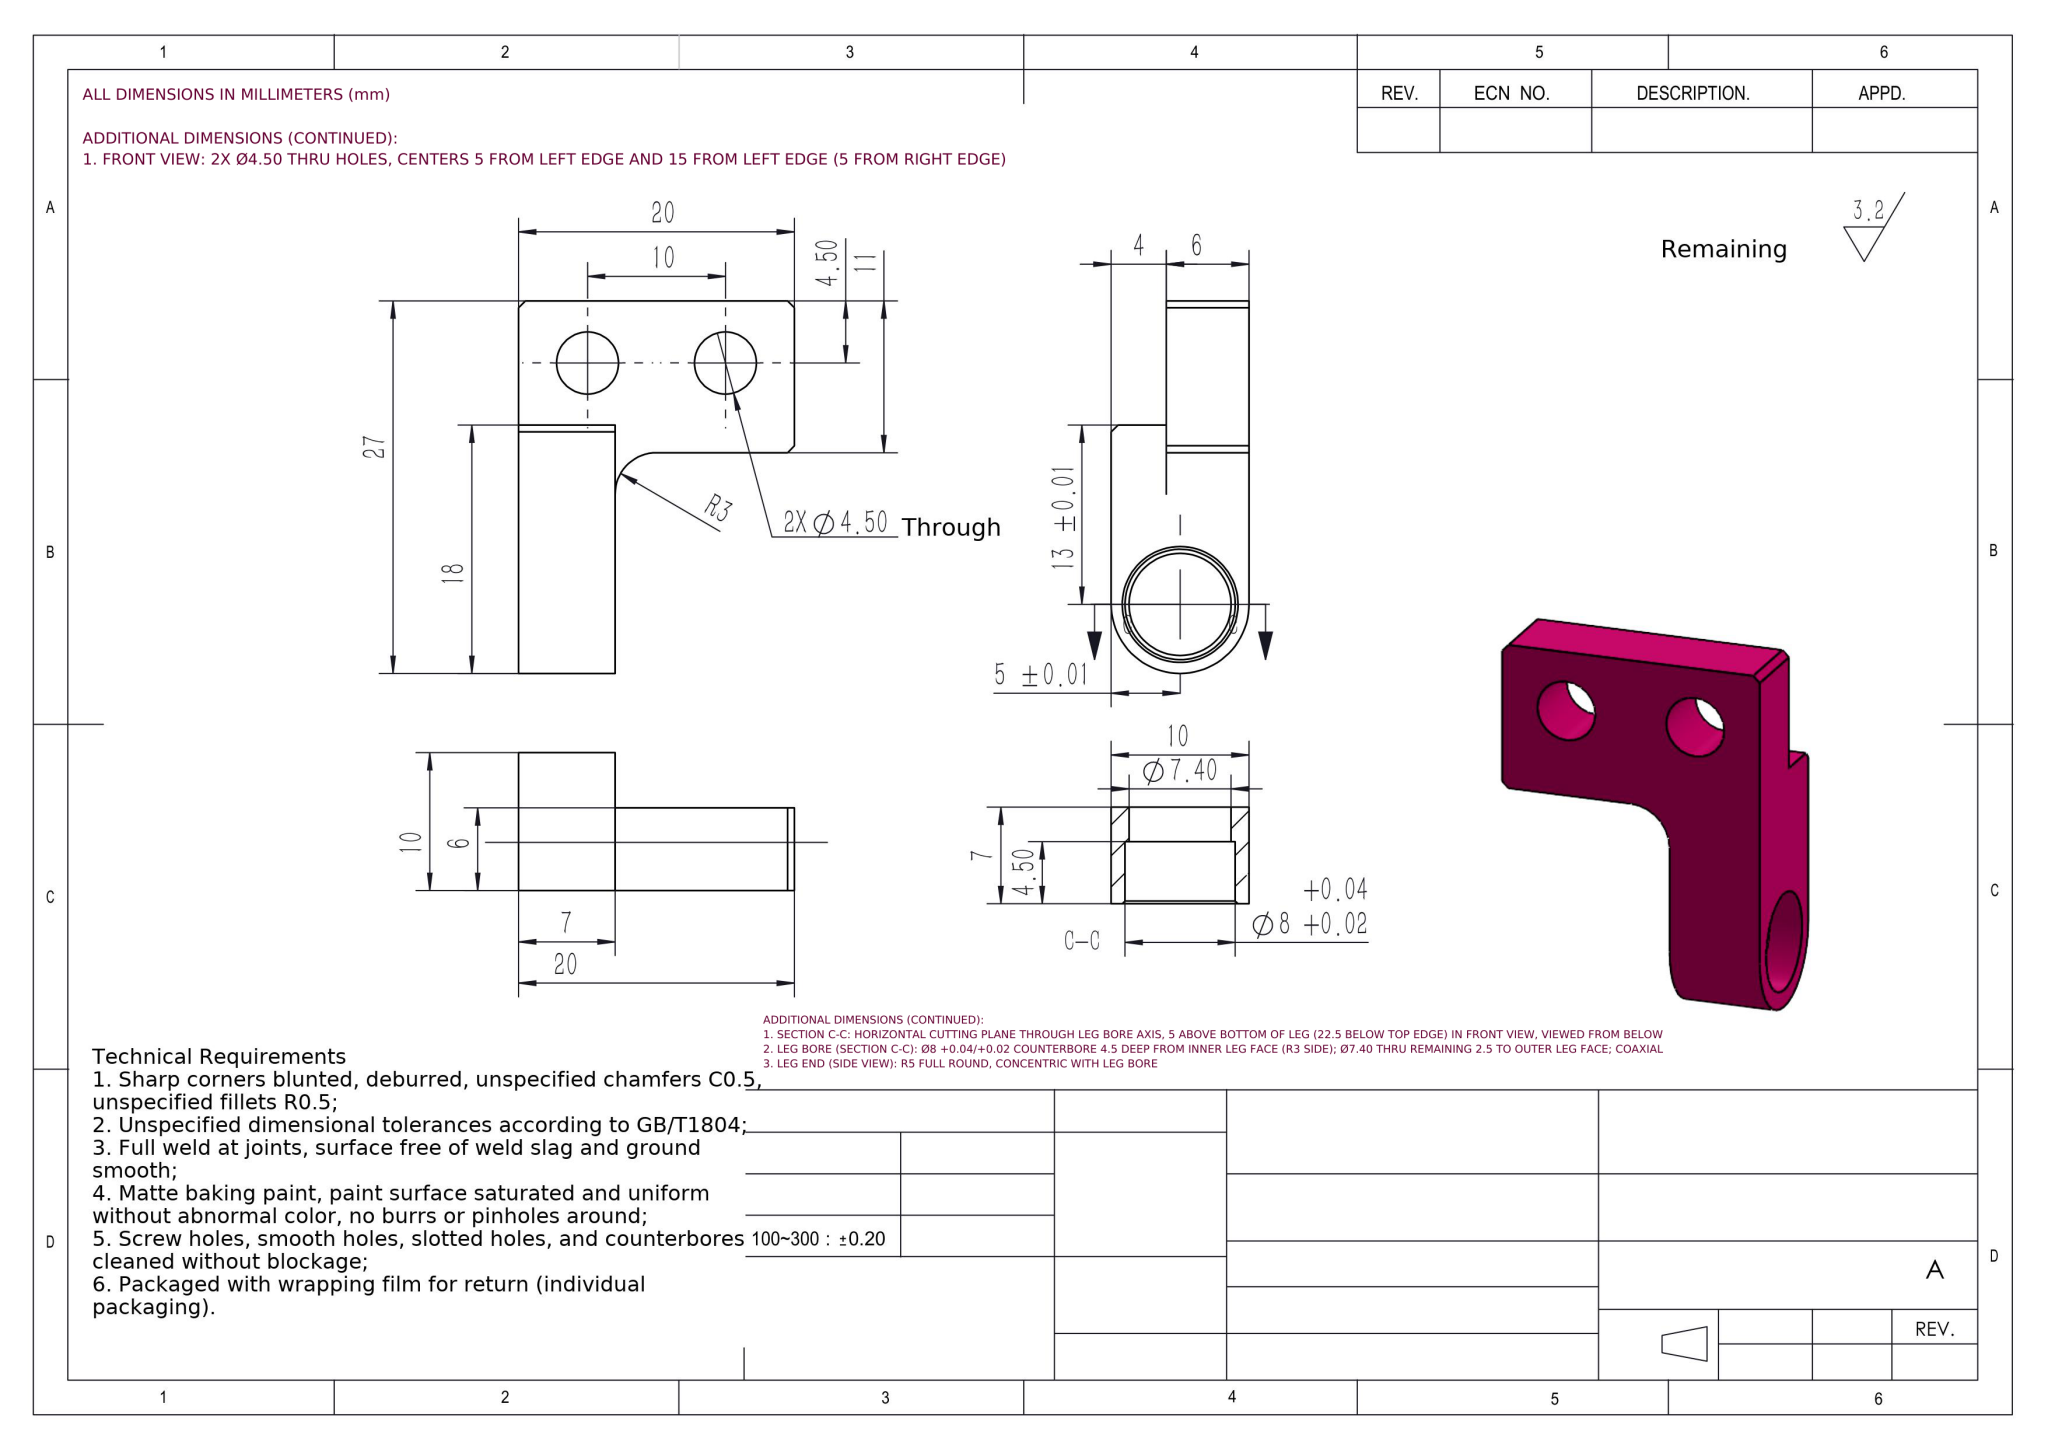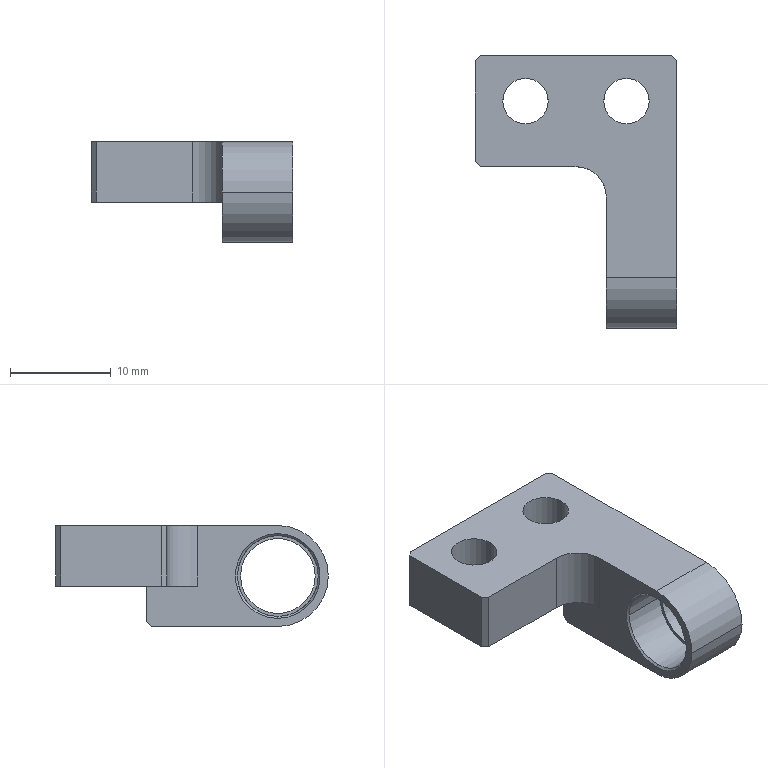Part | NX | mm | 1 solid | 27 faces | box 20 x 27 x 10 mm | volume 1904 mm3 | plane 14 | cylinder 11 | cone 2 | commonest cylinder face diameters 4.5 x4 8 x2 7.4 x2 10 x2 6 x1
STEP:
#1=COLOUR_RGB('',0.7922,0.8196,0.9333);
#2=FILL_AREA_STYLE_COLOUR('',#1);
#3=FILL_AREA_STYLE('',(#2));
#4=SURFACE_STYLE_FILL_AREA(#3);
#5=SURFACE_SIDE_STYLE('',(#4));
#6=SURFACE_STYLE_USAGE(.BOTH.,#5);
#7=PRESENTATION_STYLE_ASSIGNMENT((#6));
#8=CARTESIAN_POINT('',(3.2,-17.5,-6.));
#9=VERTEX_POINT('',#8);
#10=CARTESIAN_POINT('',(3.2,-21.5,-2.));
#11=VERTEX_POINT('',#10);
#12=CARTESIAN_POINT('',(3.2,-17.5,-2.));
#13=DIRECTION('',(-1.,0.,0.));
#14=DIRECTION('',(0.,0.,-1.));
#15=AXIS2_PLACEMENT_3D('',#12,#13,#14);
#16=CIRCLE('',#15,4.);
#17=EDGE_CURVE('',#9,#11,#16,.T.);
#18=ORIENTED_EDGE('',*,*,#17,.F.);
#19=CARTESIAN_POINT('',(3.,-17.5,-6.2));
#20=VERTEX_POINT('',#19);
#21=CARTESIAN_POINT('',(3.2,-17.5,-6.));
#22=DIRECTION('',(-0.7071,0.,-0.7071));
#23=VECTOR('',#22,1000.);
#24=LINE('',#21,#23);
#25=EDGE_CURVE('',#9,#20,#24,.T.);
#26=ORIENTED_EDGE('',*,*,#25,.T.);
#27=CARTESIAN_POINT('',(3.,-17.5,2.2));
#28=VERTEX_POINT('',#27);
#29=CARTESIAN_POINT('',(3.,-17.5,-2.));
#30=DIRECTION('',(1.,0.,0.));
#31=DIRECTION('',(-0.,1.,0.));
#32=AXIS2_PLACEMENT_3D('',#29,#30,#31);
#33=CIRCLE('',#32,4.2);
#34=EDGE_CURVE('',#28,#20,#33,.T.);
#35=ORIENTED_EDGE('',*,*,#34,.F.);
#36=CARTESIAN_POINT('',(3.2,-17.5,2.));
#37=VERTEX_POINT('',#36);
#38=CARTESIAN_POINT('',(3.2,-17.5,2.));
#39=DIRECTION('',(-0.7071,0.,0.7071));
#40=VECTOR('',#39,1000.);
#41=LINE('',#38,#40);
#42=EDGE_CURVE('',#37,#28,#41,.T.);
#43=ORIENTED_EDGE('',*,*,#42,.F.);
#44=CARTESIAN_POINT('',(3.2,-17.5,-2.));
#45=DIRECTION('',(-1.,0.,0.));
#46=DIRECTION('',(0.,0.,-1.));
#47=AXIS2_PLACEMENT_3D('',#44,#45,#46);
#48=CIRCLE('',#47,4.);
#49=EDGE_CURVE('',#11,#37,#48,.T.);
#50=ORIENTED_EDGE('',*,*,#49,.F.);
#51=EDGE_LOOP('',(#18,#26,#35,#43,#50));
#52=FACE_OUTER_BOUND('',#51,.T.);
#53=CARTESIAN_POINT('',(3.2,-17.5,-2.));
#54=DIRECTION('',(-1.,0.,0.));
#55=DIRECTION('',(0.,0.,1.));
#56=AXIS2_PLACEMENT_3D('',#53,#54,#55);
#57=CONICAL_SURFACE('',#56,4.,0.7854);
#58=ADVANCED_FACE('',(#52),#57,.F.);
#59=CARTESIAN_POINT('',(-2.75,0.,3.));
#60=VERTEX_POINT('',#59);
#61=CARTESIAN_POINT('',(-7.25,0.,3.));
#62=VERTEX_POINT('',#61);
#63=CARTESIAN_POINT('',(-5.,0.,3.));
#64=DIRECTION('',(0.,0.,-1.));
#65=DIRECTION('',(-1.,0.,0.));
#66=AXIS2_PLACEMENT_3D('',#63,#64,#65);
#67=CIRCLE('',#66,2.25);
#68=EDGE_CURVE('',#60,#62,#67,.T.);
#69=ORIENTED_EDGE('',*,*,#68,.F.);
#70=CARTESIAN_POINT('',(-2.75,0.,-3.));
#71=VERTEX_POINT('',#70);
#72=CARTESIAN_POINT('',(-2.75,0.,3.));
#73=DIRECTION('',(0.,0.,-1.));
#74=VECTOR('',#73,1000.);
#75=LINE('',#72,#74);
#76=EDGE_CURVE('',#60,#71,#75,.T.);
#77=ORIENTED_EDGE('',*,*,#76,.T.);
#78=CARTESIAN_POINT('',(-7.25,0.,-3.));
#79=VERTEX_POINT('',#78);
#80=CARTESIAN_POINT('',(-5.,0.,-3.));
#81=DIRECTION('',(0.,0.,-1.));
#82=DIRECTION('',(-1.,0.,0.));
#83=AXIS2_PLACEMENT_3D('',#80,#81,#82);
#84=CIRCLE('',#83,2.25);
#85=EDGE_CURVE('',#71,#79,#84,.T.);
#86=ORIENTED_EDGE('',*,*,#85,.T.);
#87=CARTESIAN_POINT('',(-7.25,0.,3.));
#88=DIRECTION('',(0.,0.,-1.));
#89=VECTOR('',#88,1000.);
#90=LINE('',#87,#89);
#91=EDGE_CURVE('',#62,#79,#90,.T.);
#92=ORIENTED_EDGE('',*,*,#91,.F.);
#93=EDGE_LOOP('',(#69,#77,#86,#92));
#94=FACE_OUTER_BOUND('',#93,.T.);
#95=CARTESIAN_POINT('',(-5.,0.,3.));
#96=DIRECTION('',(0.,0.,-1.));
#97=DIRECTION('',(-1.,0.,0.));
#98=AXIS2_PLACEMENT_3D('',#95,#96,#97);
#99=CYLINDRICAL_SURFACE('',#98,2.25);
#100=ADVANCED_FACE('',(#94),#99,.F.);
#101=CARTESIAN_POINT('',(7.25,-0.,3.));
#102=VERTEX_POINT('',#101);
#103=CARTESIAN_POINT('',(2.75,-0.,3.));
#104=VERTEX_POINT('',#103);
#105=CARTESIAN_POINT('',(5.,-0.,3.));
#106=DIRECTION('',(0.,0.,-1.));
#107=DIRECTION('',(-1.,0.,0.));
#108=AXIS2_PLACEMENT_3D('',#105,#106,#107);
#109=CIRCLE('',#108,2.25);
#110=EDGE_CURVE('',#102,#104,#109,.T.);
#111=ORIENTED_EDGE('',*,*,#110,.F.);
#112=CARTESIAN_POINT('',(7.25,-0.,-3.));
#113=VERTEX_POINT('',#112);
#114=CARTESIAN_POINT('',(7.25,-0.,3.));
#115=DIRECTION('',(0.,0.,-1.));
#116=VECTOR('',#115,1000.);
#117=LINE('',#114,#116);
#118=EDGE_CURVE('',#102,#113,#117,.T.);
#119=ORIENTED_EDGE('',*,*,#118,.T.);
#120=CARTESIAN_POINT('',(2.75,-0.,-3.));
#121=VERTEX_POINT('',#120);
#122=CARTESIAN_POINT('',(5.,-0.,-3.));
#123=DIRECTION('',(0.,0.,-1.));
#124=DIRECTION('',(-1.,0.,0.));
#125=AXIS2_PLACEMENT_3D('',#122,#123,#124);
#126=CIRCLE('',#125,2.25);
#127=EDGE_CURVE('',#113,#121,#126,.T.);
#128=ORIENTED_EDGE('',*,*,#127,.T.);
#129=CARTESIAN_POINT('',(2.75,-0.,3.));
#130=DIRECTION('',(0.,0.,-1.));
#131=VECTOR('',#130,1000.);
#132=LINE('',#129,#131);
#133=EDGE_CURVE('',#104,#121,#132,.T.);
#134=ORIENTED_EDGE('',*,*,#133,.F.);
#135=EDGE_LOOP('',(#111,#119,#128,#134));
#136=FACE_OUTER_BOUND('',#135,.T.);
#137=CARTESIAN_POINT('',(5.,-0.,3.));
#138=DIRECTION('',(0.,0.,-1.));
#139=DIRECTION('',(-1.,0.,0.));
#140=AXIS2_PLACEMENT_3D('',#137,#138,#139);
#141=CYLINDRICAL_SURFACE('',#140,2.25);
#142=ADVANCED_FACE('',(#136),#141,.F.);
#143=CARTESIAN_POINT('',(7.5,-13.5,-2.));
#144=VERTEX_POINT('',#143);
#145=CARTESIAN_POINT('',(7.5,-21.5,-2.));
#146=VERTEX_POINT('',#145);
#147=CARTESIAN_POINT('',(7.5,-17.5,-2.));
#148=DIRECTION('',(-1.,-0.,0.));
#149=DIRECTION('',(0.,-1.,0.));
#150=AXIS2_PLACEMENT_3D('',#147,#148,#149);
#151=CIRCLE('',#150,4.);
#152=EDGE_CURVE('',#144,#146,#151,.T.);
#153=ORIENTED_EDGE('',*,*,#152,.F.);
#154=CARTESIAN_POINT('',(3.2,-13.5,-2.));
#155=VERTEX_POINT('',#154);
#156=CARTESIAN_POINT('',(7.5,-13.5,-2.));
#157=DIRECTION('',(-1.,-0.,0.));
#158=VECTOR('',#157,1000.);
#159=LINE('',#156,#158);
#160=EDGE_CURVE('',#144,#155,#159,.T.);
#161=ORIENTED_EDGE('',*,*,#160,.T.);
#162=CARTESIAN_POINT('',(3.2,-17.5,-2.));
#163=DIRECTION('',(-1.,0.,0.));
#164=DIRECTION('',(0.,0.,-1.));
#165=AXIS2_PLACEMENT_3D('',#162,#163,#164);
#166=CIRCLE('',#165,4.);
#167=EDGE_CURVE('',#155,#9,#166,.T.);
#168=ORIENTED_EDGE('',*,*,#167,.T.);
#169=ORIENTED_EDGE('',*,*,#17,.T.);
#170=CARTESIAN_POINT('',(7.5,-21.5,-2.));
#171=DIRECTION('',(-1.,-0.,0.));
#172=VECTOR('',#171,1000.);
#173=LINE('',#170,#172);
#174=EDGE_CURVE('',#146,#11,#173,.T.);
#175=ORIENTED_EDGE('',*,*,#174,.F.);
#176=EDGE_LOOP('',(#153,#161,#168,#169,#175));
#177=FACE_OUTER_BOUND('',#176,.T.);
#178=CARTESIAN_POINT('',(7.5,-17.5,-2.));
#179=DIRECTION('',(-1.,-0.,0.));
#180=DIRECTION('',(0.,-1.,0.));
#181=AXIS2_PLACEMENT_3D('',#178,#179,#180);
#182=CYLINDRICAL_SURFACE('',#181,4.);
#183=ADVANCED_FACE('',(#177),#182,.F.);
#184=CARTESIAN_POINT('',(10.,-13.8,-2.));
#185=VERTEX_POINT('',#184);
#186=CARTESIAN_POINT('',(10.,-21.2,-2.));
#187=VERTEX_POINT('',#186);
#188=CARTESIAN_POINT('',(10.,-17.5,-2.));
#189=DIRECTION('',(-1.,-0.,0.));
#190=DIRECTION('',(0.,-1.,0.));
#191=AXIS2_PLACEMENT_3D('',#188,#189,#190);
#192=CIRCLE('',#191,3.7);
#193=EDGE_CURVE('',#185,#187,#192,.T.);
#194=ORIENTED_EDGE('',*,*,#193,.F.);
#195=CARTESIAN_POINT('',(7.5,-13.8,-2.));
#196=VERTEX_POINT('',#195);
#197=CARTESIAN_POINT('',(10.,-13.8,-2.));
#198=DIRECTION('',(-1.,-0.,0.));
#199=VECTOR('',#198,1000.);
#200=LINE('',#197,#199);
#201=EDGE_CURVE('',#185,#196,#200,.T.);
#202=ORIENTED_EDGE('',*,*,#201,.T.);
#203=CARTESIAN_POINT('',(7.5,-21.2,-2.));
#204=VERTEX_POINT('',#203);
#205=CARTESIAN_POINT('',(7.5,-17.5,-2.));
#206=DIRECTION('',(1.,0.,0.));
#207=DIRECTION('',(0.,-1.,0.));
#208=AXIS2_PLACEMENT_3D('',#205,#206,#207);
#209=CIRCLE('',#208,3.7);
#210=EDGE_CURVE('',#204,#196,#209,.T.);
#211=ORIENTED_EDGE('',*,*,#210,.F.);
#212=CARTESIAN_POINT('',(10.,-21.2,-2.));
#213=DIRECTION('',(-1.,-0.,0.));
#214=VECTOR('',#213,1000.);
#215=LINE('',#212,#214);
#216=EDGE_CURVE('',#187,#204,#215,.T.);
#217=ORIENTED_EDGE('',*,*,#216,.F.);
#218=EDGE_LOOP('',(#194,#202,#211,#217));
#219=FACE_OUTER_BOUND('',#218,.T.);
#220=CARTESIAN_POINT('',(10.,-17.5,-2.));
#221=DIRECTION('',(-1.,-0.,0.));
#222=DIRECTION('',(0.,-1.,0.));
#223=AXIS2_PLACEMENT_3D('',#220,#221,#222);
#224=CYLINDRICAL_SURFACE('',#223,3.7);
#225=ADVANCED_FACE('',(#219),#224,.F.);
#226=ORIENTED_EDGE('',*,*,#34,.T.);
#227=CARTESIAN_POINT('',(3.,-17.5,-2.));
#228=DIRECTION('',(1.,0.,0.));
#229=DIRECTION('',(-0.,1.,0.));
#230=AXIS2_PLACEMENT_3D('',#227,#228,#229);
#231=CIRCLE('',#230,4.2);
#232=EDGE_CURVE('',#20,#28,#231,.T.);
#233=ORIENTED_EDGE('',*,*,#232,.T.);
#234=EDGE_LOOP('',(#226,#233));
#235=FACE_BOUND('',#234,.T.);
#236=CARTESIAN_POINT('',(3.,-9.5,3.));
#237=VERTEX_POINT('',#236);
#238=CARTESIAN_POINT('',(3.,-17.5,3.));
#239=VERTEX_POINT('',#238);
#240=CARTESIAN_POINT('',(3.,-4.5,3.));
#241=DIRECTION('',(0.,-1.,-0.));
#242=VECTOR('',#241,1000.);
#243=LINE('',#240,#242);
#244=EDGE_CURVE('',#237,#239,#243,.T.);
#245=ORIENTED_EDGE('',*,*,#244,.F.);
#246=CARTESIAN_POINT('',(3.,-9.5,-3.));
#247=VERTEX_POINT('',#246);
#248=CARTESIAN_POINT('',(3.,-9.5,-3.));
#249=DIRECTION('',(0.,0.,-1.));
#250=VECTOR('',#249,1000.);
#251=LINE('',#248,#250);
#252=EDGE_CURVE('',#237,#247,#251,.T.);
#253=ORIENTED_EDGE('',*,*,#252,.T.);
#254=CARTESIAN_POINT('',(3.,-4.5,-3.));
#255=VERTEX_POINT('',#254);
#256=CARTESIAN_POINT('',(3.,-6.5,-3.));
#257=DIRECTION('',(0.,1.,0.));
#258=VECTOR('',#257,1000.);
#259=LINE('',#256,#258);
#260=EDGE_CURVE('',#247,#255,#259,.T.);
#261=ORIENTED_EDGE('',*,*,#260,.T.);
#262=CARTESIAN_POINT('',(3.,-4.5,-6.5));
#263=VERTEX_POINT('',#262);
#264=CARTESIAN_POINT('',(3.,-4.5,3.));
#265=DIRECTION('',(0.,0.,1.));
#266=VECTOR('',#265,1000.);
#267=LINE('',#264,#266);
#268=EDGE_CURVE('',#263,#255,#267,.T.);
#269=ORIENTED_EDGE('',*,*,#268,.F.);
#270=CARTESIAN_POINT('',(3.,-5.,-7.));
#271=VERTEX_POINT('',#270);
#272=CARTESIAN_POINT('',(3.,-5.,-7.));
#273=DIRECTION('',(0.,-0.7071,-0.7071));
#274=VECTOR('',#273,1000.);
#275=LINE('',#272,#274);
#276=EDGE_CURVE('',#263,#271,#275,.T.);
#277=ORIENTED_EDGE('',*,*,#276,.T.);
#278=CARTESIAN_POINT('',(3.,-17.5,-7.));
#279=VERTEX_POINT('',#278);
#280=CARTESIAN_POINT('',(3.,-4.5,-7.));
#281=DIRECTION('',(-0.,1.,0.));
#282=VECTOR('',#281,1000.);
#283=LINE('',#280,#282);
#284=EDGE_CURVE('',#279,#271,#283,.T.);
#285=ORIENTED_EDGE('',*,*,#284,.F.);
#286=CARTESIAN_POINT('',(3.,-22.5,-2.));
#287=VERTEX_POINT('',#286);
#288=CARTESIAN_POINT('',(3.,-17.5,-2.));
#289=DIRECTION('',(-1.,-0.,0.));
#290=DIRECTION('',(-0.,1.,0.));
#291=AXIS2_PLACEMENT_3D('',#288,#289,#290);
#292=CIRCLE('',#291,5.);
#293=EDGE_CURVE('',#279,#287,#292,.T.);
#294=ORIENTED_EDGE('',*,*,#293,.T.);
#295=CARTESIAN_POINT('',(3.,-17.5,-2.));
#296=DIRECTION('',(-1.,-0.,0.));
#297=DIRECTION('',(-0.,1.,0.));
#298=AXIS2_PLACEMENT_3D('',#295,#296,#297);
#299=CIRCLE('',#298,5.);
#300=EDGE_CURVE('',#287,#239,#299,.T.);
#301=ORIENTED_EDGE('',*,*,#300,.T.);
#302=EDGE_LOOP('',(#245,#253,#261,#269,#277,#285,#294,#301));
#303=FACE_OUTER_BOUND('',#302,.T.);
#304=CARTESIAN_POINT('',(3.,0.,0.));
#305=DIRECTION('',(1.,0.,0.));
#306=DIRECTION('',(-0.,1.,0.));
#307=AXIS2_PLACEMENT_3D('',#304,#305,#306);
#308=PLANE('',#307);
#309=ADVANCED_FACE('',(#235,#303),#308,.F.);
#310=ORIENTED_EDGE('',*,*,#201,.F.);
#311=CARTESIAN_POINT('',(10.,-17.5,-2.));
#312=DIRECTION('',(-1.,-0.,0.));
#313=DIRECTION('',(0.,-1.,0.));
#314=AXIS2_PLACEMENT_3D('',#311,#312,#313);
#315=CIRCLE('',#314,3.7);
#316=EDGE_CURVE('',#187,#185,#315,.T.);
#317=ORIENTED_EDGE('',*,*,#316,.F.);
#318=ORIENTED_EDGE('',*,*,#216,.T.);
#319=CARTESIAN_POINT('',(7.5,-17.5,-2.));
#320=DIRECTION('',(1.,0.,0.));
#321=DIRECTION('',(0.,-1.,0.));
#322=AXIS2_PLACEMENT_3D('',#319,#320,#321);
#323=CIRCLE('',#322,3.7);
#324=EDGE_CURVE('',#196,#204,#323,.T.);
#325=ORIENTED_EDGE('',*,*,#324,.F.);
#326=EDGE_LOOP('',(#310,#317,#318,#325));
#327=FACE_OUTER_BOUND('',#326,.T.);
#328=CARTESIAN_POINT('',(10.,-17.5,-2.));
#329=DIRECTION('',(-1.,-0.,0.));
#330=DIRECTION('',(0.,-1.,0.));
#331=AXIS2_PLACEMENT_3D('',#328,#329,#330);
#332=CYLINDRICAL_SURFACE('',#331,3.7);
#333=ADVANCED_FACE('',(#327),#332,.F.);
#334=ORIENTED_EDGE('',*,*,#316,.T.);
#335=ORIENTED_EDGE('',*,*,#193,.T.);
#336=EDGE_LOOP('',(#334,#335));
#337=FACE_BOUND('',#336,.T.);
#338=CARTESIAN_POINT('',(10.,-17.5,-7.));
#339=VERTEX_POINT('',#338);
#340=CARTESIAN_POINT('',(10.,-5.,-7.));
#341=VERTEX_POINT('',#340);
#342=CARTESIAN_POINT('',(10.,-4.5,-7.));
#343=DIRECTION('',(-0.,1.,0.));
#344=VECTOR('',#343,1000.);
#345=LINE('',#342,#344);
#346=EDGE_CURVE('',#339,#341,#345,.T.);
#347=ORIENTED_EDGE('',*,*,#346,.T.);
#348=CARTESIAN_POINT('',(10.,-4.5,-6.5));
#349=VERTEX_POINT('',#348);
#350=CARTESIAN_POINT('',(10.,-5.,-7.));
#351=DIRECTION('',(0.,0.7071,0.7071));
#352=VECTOR('',#351,1000.);
#353=LINE('',#350,#352);
#354=EDGE_CURVE('',#341,#349,#353,.T.);
#355=ORIENTED_EDGE('',*,*,#354,.T.);
#356=CARTESIAN_POINT('',(10.,-4.5,-3.));
#357=VERTEX_POINT('',#356);
#358=CARTESIAN_POINT('',(10.,-4.5,3.));
#359=DIRECTION('',(0.,0.,1.));
#360=VECTOR('',#359,1000.);
#361=LINE('',#358,#360);
#362=EDGE_CURVE('',#349,#357,#361,.T.);
#363=ORIENTED_EDGE('',*,*,#362,.T.);
#364=CARTESIAN_POINT('',(10.,4.,-3.));
#365=VERTEX_POINT('',#364);
#366=CARTESIAN_POINT('',(10.,4.5,-3.));
#367=DIRECTION('',(0.,1.,0.));
#368=VECTOR('',#367,1000.);
#369=LINE('',#366,#368);
#370=EDGE_CURVE('',#357,#365,#369,.T.);
#371=ORIENTED_EDGE('',*,*,#370,.T.);
#372=CARTESIAN_POINT('',(10.,4.,3.));
#373=VERTEX_POINT('',#372);
#374=CARTESIAN_POINT('',(10.,4.,3.));
#375=DIRECTION('',(0.,0.,1.));
#376=VECTOR('',#375,1000.);
#377=LINE('',#374,#376);
#378=EDGE_CURVE('',#365,#373,#377,.T.);
#379=ORIENTED_EDGE('',*,*,#378,.T.);
#380=CARTESIAN_POINT('',(10.,-17.5,3.));
#381=VERTEX_POINT('',#380);
#382=CARTESIAN_POINT('',(10.,4.5,3.));
#383=DIRECTION('',(0.,1.,0.));
#384=VECTOR('',#383,1000.);
#385=LINE('',#382,#384);
#386=EDGE_CURVE('',#381,#373,#385,.T.);
#387=ORIENTED_EDGE('',*,*,#386,.F.);
#388=CARTESIAN_POINT('',(10.,-22.5,-2.));
#389=VERTEX_POINT('',#388);
#390=CARTESIAN_POINT('',(10.,-17.5,-2.));
#391=DIRECTION('',(1.,0.,0.));
#392=DIRECTION('',(0.,0.,1.));
#393=AXIS2_PLACEMENT_3D('',#390,#391,#392);
#394=CIRCLE('',#393,5.);
#395=EDGE_CURVE('',#381,#389,#394,.T.);
#396=ORIENTED_EDGE('',*,*,#395,.T.);
#397=CARTESIAN_POINT('',(10.,-17.5,-2.));
#398=DIRECTION('',(1.,0.,0.));
#399=DIRECTION('',(0.,0.,1.));
#400=AXIS2_PLACEMENT_3D('',#397,#398,#399);
#401=CIRCLE('',#400,5.);
#402=EDGE_CURVE('',#389,#339,#401,.T.);
#403=ORIENTED_EDGE('',*,*,#402,.T.);
#404=EDGE_LOOP('',(#347,#355,#363,#371,#379,#387,#396,#403));
#405=FACE_OUTER_BOUND('',#404,.T.);
#406=CARTESIAN_POINT('',(10.,4.5,3.));
#407=DIRECTION('',(-1.,0.,0.));
#408=DIRECTION('',(0.,0.,1.));
#409=AXIS2_PLACEMENT_3D('',#406,#407,#408);
#410=PLANE('',#409);
#411=ADVANCED_FACE('',(#337,#405),#410,.F.);
#412=CARTESIAN_POINT('',(9.5,4.5,3.));
#413=VERTEX_POINT('',#412);
#414=CARTESIAN_POINT('',(-9.5,4.5,3.));
#415=VERTEX_POINT('',#414);
#416=CARTESIAN_POINT('',(-10.,4.5,3.));
#417=DIRECTION('',(-1.,0.,0.));
#418=VECTOR('',#417,1000.);
#419=LINE('',#416,#418);
#420=EDGE_CURVE('',#413,#415,#419,.T.);
#421=ORIENTED_EDGE('',*,*,#420,.F.);
#422=CARTESIAN_POINT('',(9.5,4.5,-3.));
#423=VERTEX_POINT('',#422);
#424=CARTESIAN_POINT('',(9.5,4.5,3.));
#425=DIRECTION('',(0.,0.,-1.));
#426=VECTOR('',#425,1000.);
#427=LINE('',#424,#426);
#428=EDGE_CURVE('',#413,#423,#427,.T.);
#429=ORIENTED_EDGE('',*,*,#428,.T.);
#430=CARTESIAN_POINT('',(-9.5,4.5,-3.));
#431=VERTEX_POINT('',#430);
#432=CARTESIAN_POINT('',(-10.,4.5,-3.));
#433=DIRECTION('',(-1.,0.,0.));
#434=VECTOR('',#433,1000.);
#435=LINE('',#432,#434);
#436=EDGE_CURVE('',#423,#431,#435,.T.);
#437=ORIENTED_EDGE('',*,*,#436,.T.);
#438=CARTESIAN_POINT('',(-9.5,4.5,3.));
#439=DIRECTION('',(0.,0.,1.));
#440=VECTOR('',#439,1000.);
#441=LINE('',#438,#440);
#442=EDGE_CURVE('',#431,#415,#441,.T.);
#443=ORIENTED_EDGE('',*,*,#442,.T.);
#444=EDGE_LOOP('',(#421,#429,#437,#443));
#445=FACE_OUTER_BOUND('',#444,.T.);
#446=CARTESIAN_POINT('',(-10.,4.5,3.));
#447=DIRECTION('',(0.,-1.,0.));
#448=DIRECTION('',(0.,0.,-1.));
#449=AXIS2_PLACEMENT_3D('',#446,#447,#448);
#450=PLANE('',#449);
#451=ADVANCED_FACE('',(#445),#450,.F.);
#452=CARTESIAN_POINT('',(-10.,4.,-3.));
#453=VERTEX_POINT('',#452);
#454=CARTESIAN_POINT('',(-10.,-6.,-3.));
#455=VERTEX_POINT('',#454);
#456=CARTESIAN_POINT('',(-10.,4.5,-3.));
#457=DIRECTION('',(0.,-1.,0.));
#458=VECTOR('',#457,1000.);
#459=LINE('',#456,#458);
#460=EDGE_CURVE('',#453,#455,#459,.T.);
#461=ORIENTED_EDGE('',*,*,#460,.T.);
#462=CARTESIAN_POINT('',(-10.,-6.,3.));
#463=VERTEX_POINT('',#462);
#464=CARTESIAN_POINT('',(-10.,-6.,3.));
#465=DIRECTION('',(0.,0.,1.));
#466=VECTOR('',#465,1000.);
#467=LINE('',#464,#466);
#468=EDGE_CURVE('',#455,#463,#467,.T.);
#469=ORIENTED_EDGE('',*,*,#468,.T.);
#470=CARTESIAN_POINT('',(-10.,4.,3.));
#471=VERTEX_POINT('',#470);
#472=CARTESIAN_POINT('',(-10.,4.5,3.));
#473=DIRECTION('',(0.,-1.,0.));
#474=VECTOR('',#473,1000.);
#475=LINE('',#472,#474);
#476=EDGE_CURVE('',#471,#463,#475,.T.);
#477=ORIENTED_EDGE('',*,*,#476,.F.);
#478=CARTESIAN_POINT('',(-10.,4.,3.));
#479=DIRECTION('',(0.,0.,-1.));
#480=VECTOR('',#479,1000.);
#481=LINE('',#478,#480);
#482=EDGE_CURVE('',#471,#453,#481,.T.);
#483=ORIENTED_EDGE('',*,*,#482,.T.);
#484=EDGE_LOOP('',(#461,#469,#477,#483));
#485=FACE_OUTER_BOUND('',#484,.T.);
#486=CARTESIAN_POINT('',(-10.,4.5,3.));
#487=DIRECTION('',(1.,0.,0.));
#488=DIRECTION('',(0.,0.,-1.));
#489=AXIS2_PLACEMENT_3D('',#486,#487,#488);
#490=PLANE('',#489);
#491=ADVANCED_FACE('',(#485),#490,.F.);
#492=CARTESIAN_POINT('',(-5.,0.,3.));
#493=DIRECTION('',(0.,0.,-1.));
#494=DIRECTION('',(-1.,0.,0.));
#495=AXIS2_PLACEMENT_3D('',#492,#493,#494);
#496=CIRCLE('',#495,2.25);
#497=EDGE_CURVE('',#62,#60,#496,.T.);
#498=ORIENTED_EDGE('',*,*,#497,.T.);
#499=ORIENTED_EDGE('',*,*,#68,.T.);
#500=EDGE_LOOP('',(#498,#499));
#501=FACE_BOUND('',#500,.T.);
#502=CARTESIAN_POINT('',(5.,-0.,3.));
#503=DIRECTION('',(0.,0.,-1.));
#504=DIRECTION('',(-1.,0.,0.));
#505=AXIS2_PLACEMENT_3D('',#502,#503,#504);
#506=CIRCLE('',#505,2.25);
#507=EDGE_CURVE('',#104,#102,#506,.T.);
#508=ORIENTED_EDGE('',*,*,#507,.T.);
#509=ORIENTED_EDGE('',*,*,#110,.T.);
#510=EDGE_LOOP('',(#508,#509));
#511=FACE_BOUND('',#510,.T.);
#512=ORIENTED_EDGE('',*,*,#476,.T.);
#513=CARTESIAN_POINT('',(-9.5,-6.5,3.));
#514=VERTEX_POINT('',#513);
#515=CARTESIAN_POINT('',(-8.,-8.,3.));
#516=DIRECTION('',(0.7071,-0.7071,0.));
#517=VECTOR('',#516,1000.);
#518=LINE('',#515,#517);
#519=EDGE_CURVE('',#463,#514,#518,.T.);
#520=ORIENTED_EDGE('',*,*,#519,.T.);
#521=CARTESIAN_POINT('',(0.,-6.5,3.));
#522=VERTEX_POINT('',#521);
#523=CARTESIAN_POINT('',(3.,-6.5,3.));
#524=DIRECTION('',(-1.,0.,-0.));
#525=VECTOR('',#524,1000.);
#526=LINE('',#523,#525);
#527=EDGE_CURVE('',#522,#514,#526,.T.);
#528=ORIENTED_EDGE('',*,*,#527,.F.);
#529=CARTESIAN_POINT('',(0.,-9.5,3.));
#530=DIRECTION('',(0.,0.,-1.));
#531=DIRECTION('',(1.,0.,0.));
#532=AXIS2_PLACEMENT_3D('',#529,#530,#531);
#533=CIRCLE('',#532,3.);
#534=EDGE_CURVE('',#522,#237,#533,.T.);
#535=ORIENTED_EDGE('',*,*,#534,.T.);
#536=ORIENTED_EDGE('',*,*,#244,.T.);
#537=CARTESIAN_POINT('',(0.,-17.5,3.));
#538=DIRECTION('',(1.,0.,0.));
#539=VECTOR('',#538,1000.);
#540=LINE('',#537,#539);
#541=EDGE_CURVE('',#239,#381,#540,.T.);
#542=ORIENTED_EDGE('',*,*,#541,.T.);
#543=ORIENTED_EDGE('',*,*,#386,.T.);
#544=CARTESIAN_POINT('',(7.,7.,3.));
#545=DIRECTION('',(-0.7071,0.7071,0.));
#546=VECTOR('',#545,1000.);
#547=LINE('',#544,#546);
#548=EDGE_CURVE('',#373,#413,#547,.T.);
#549=ORIENTED_EDGE('',*,*,#548,.T.);
#550=ORIENTED_EDGE('',*,*,#420,.T.);
#551=CARTESIAN_POINT('',(-7.,7.,3.));
#552=DIRECTION('',(-0.7071,-0.7071,0.));
#553=VECTOR('',#552,1000.);
#554=LINE('',#551,#553);
#555=EDGE_CURVE('',#415,#471,#554,.T.);
#556=ORIENTED_EDGE('',*,*,#555,.T.);
#557=EDGE_LOOP('',(#512,#520,#528,#535,#536,#542,#543,#549,#550,#556));
#558=FACE_OUTER_BOUND('',#557,.T.);
#559=CARTESIAN_POINT('',(0.,0.,3.));
#560=DIRECTION('',(0.,0.,1.));
#561=DIRECTION('',(1.,0.,0.));
#562=AXIS2_PLACEMENT_3D('',#559,#560,#561);
#563=PLANE('',#562);
#564=ADVANCED_FACE('',(#501,#511,#558),#563,.T.);
#565=CARTESIAN_POINT('',(-5.,0.,-3.));
#566=DIRECTION('',(0.,0.,-1.));
#567=DIRECTION('',(-1.,0.,0.));
#568=AXIS2_PLACEMENT_3D('',#565,#566,#567);
#569=CIRCLE('',#568,2.25);
#570=EDGE_CURVE('',#79,#71,#569,.T.);
#571=ORIENTED_EDGE('',*,*,#570,.F.);
#572=ORIENTED_EDGE('',*,*,#85,.F.);
#573=EDGE_LOOP('',(#571,#572));
#574=FACE_BOUND('',#573,.T.);
#575=CARTESIAN_POINT('',(5.,-0.,-3.));
#576=DIRECTION('',(0.,0.,-1.));
#577=DIRECTION('',(-1.,0.,0.));
#578=AXIS2_PLACEMENT_3D('',#575,#576,#577);
#579=CIRCLE('',#578,2.25);
#580=EDGE_CURVE('',#121,#113,#579,.T.);
#581=ORIENTED_EDGE('',*,*,#580,.F.);
#582=ORIENTED_EDGE('',*,*,#127,.F.);
#583=EDGE_LOOP('',(#581,#582));
#584=FACE_BOUND('',#583,.T.);
#585=CARTESIAN_POINT('',(-9.5,-6.5,-3.));
#586=VERTEX_POINT('',#585);
#587=CARTESIAN_POINT('',(0.,-6.5,-3.));
#588=VERTEX_POINT('',#587);
#589=CARTESIAN_POINT('',(3.,-6.5,-3.));
#590=DIRECTION('',(1.,0.,0.));
#591=VECTOR('',#590,1000.);
#592=LINE('',#589,#591);
#593=EDGE_CURVE('',#586,#588,#592,.T.);
#594=ORIENTED_EDGE('',*,*,#593,.F.);
#595=CARTESIAN_POINT('',(-9.5,-6.5,-3.));
#596=DIRECTION('',(-0.7071,0.7071,0.));
#597=VECTOR('',#596,1000.);
#598=LINE('',#595,#597);
#599=EDGE_CURVE('',#586,#455,#598,.T.);
#600=ORIENTED_EDGE('',*,*,#599,.T.);
#601=ORIENTED_EDGE('',*,*,#460,.F.);
#602=CARTESIAN_POINT('',(-10.,4.,-3.));
#603=DIRECTION('',(0.7071,0.7071,0.));
#604=VECTOR('',#603,1000.);
#605=LINE('',#602,#604);
#606=EDGE_CURVE('',#453,#431,#605,.T.);
#607=ORIENTED_EDGE('',*,*,#606,.T.);
#608=ORIENTED_EDGE('',*,*,#436,.F.);
#609=CARTESIAN_POINT('',(9.5,4.5,-3.));
#610=DIRECTION('',(0.7071,-0.7071,0.));
#611=VECTOR('',#610,1000.);
#612=LINE('',#609,#611);
#613=EDGE_CURVE('',#423,#365,#612,.T.);
#614=ORIENTED_EDGE('',*,*,#613,.T.);
#615=ORIENTED_EDGE('',*,*,#370,.F.);
#616=CARTESIAN_POINT('',(-10.,-4.5,-3.));
#617=DIRECTION('',(1.,0.,0.));
#618=VECTOR('',#617,1000.);
#619=LINE('',#616,#618);
#620=EDGE_CURVE('',#255,#357,#619,.T.);
#621=ORIENTED_EDGE('',*,*,#620,.F.);
#622=ORIENTED_EDGE('',*,*,#260,.F.);
#623=CARTESIAN_POINT('',(0.,-9.5,-3.));
#624=DIRECTION('',(0.,0.,1.));
#625=DIRECTION('',(1.,0.,0.));
#626=AXIS2_PLACEMENT_3D('',#623,#624,#625);
#627=CIRCLE('',#626,3.);
#628=EDGE_CURVE('',#247,#588,#627,.T.);
#629=ORIENTED_EDGE('',*,*,#628,.T.);
#630=EDGE_LOOP('',(#594,#600,#601,#607,#608,#614,#615,#621,#622,#629));
#631=FACE_OUTER_BOUND('',#630,.T.);
#632=CARTESIAN_POINT('',(0.,0.,-3.));
#633=DIRECTION('',(0.,0.,1.));
#634=DIRECTION('',(1.,0.,0.));
#635=AXIS2_PLACEMENT_3D('',#632,#633,#634);
#636=PLANE('',#635);
#637=ADVANCED_FACE('',(#574,#584,#631),#636,.F.);
#638=ORIENTED_EDGE('',*,*,#362,.F.);
#639=CARTESIAN_POINT('',(3.,-4.5,-6.5));
#640=DIRECTION('',(-1.,-0.,0.));
#641=VECTOR('',#640,1000.);
#642=LINE('',#639,#641);
#643=EDGE_CURVE('',#349,#263,#642,.T.);
#644=ORIENTED_EDGE('',*,*,#643,.T.);
#645=ORIENTED_EDGE('',*,*,#268,.T.);
#646=ORIENTED_EDGE('',*,*,#620,.T.);
#647=EDGE_LOOP('',(#638,#644,#645,#646));
#648=FACE_OUTER_BOUND('',#647,.T.);
#649=CARTESIAN_POINT('',(3.,-4.5,3.));
#650=DIRECTION('',(-0.,1.,0.));
#651=DIRECTION('',(-1.,-0.,0.));
#652=AXIS2_PLACEMENT_3D('',#649,#650,#651);
#653=PLANE('',#652);
#654=ADVANCED_FACE('',(#648),#653,.T.);
#655=ORIENTED_EDGE('',*,*,#284,.T.);
#656=CARTESIAN_POINT('',(3.,-5.,-7.));
#657=DIRECTION('',(1.,0.,0.));
#658=VECTOR('',#657,1000.);
#659=LINE('',#656,#658);
#660=EDGE_CURVE('',#271,#341,#659,.T.);
#661=ORIENTED_EDGE('',*,*,#660,.T.);
#662=ORIENTED_EDGE('',*,*,#346,.F.);
#663=CARTESIAN_POINT('',(3.,-17.5,-7.));
#664=DIRECTION('',(-1.,-0.,0.));
#665=VECTOR('',#664,1000.);
#666=LINE('',#663,#665);
#667=EDGE_CURVE('',#339,#279,#666,.T.);
#668=ORIENTED_EDGE('',*,*,#667,.T.);
#669=EDGE_LOOP('',(#655,#661,#662,#668));
#670=FACE_OUTER_BOUND('',#669,.T.);
#671=CARTESIAN_POINT('',(3.,-4.5,-7.));
#672=DIRECTION('',(-0.,0.,-1.));
#673=DIRECTION('',(0.,1.,0.));
#674=AXIS2_PLACEMENT_3D('',#671,#672,#673);
#675=PLANE('',#674);
#676=ADVANCED_FACE('',(#670),#675,.T.);
#677=CARTESIAN_POINT('',(7.5,-17.5,-2.));
#678=DIRECTION('',(-1.,-0.,0.));
#679=DIRECTION('',(0.,-1.,0.));
#680=AXIS2_PLACEMENT_3D('',#677,#678,#679);
#681=CIRCLE('',#680,4.);
#682=EDGE_CURVE('',#146,#144,#681,.T.);
#683=ORIENTED_EDGE('',*,*,#682,.T.);
#684=ORIENTED_EDGE('',*,*,#152,.T.);
#685=EDGE_LOOP('',(#683,#684));
#686=FACE_OUTER_BOUND('',#685,.T.);
#687=ORIENTED_EDGE('',*,*,#210,.T.);
#688=ORIENTED_EDGE('',*,*,#324,.T.);
#689=EDGE_LOOP('',(#687,#688));
#690=FACE_BOUND('',#689,.T.);
#691=CARTESIAN_POINT('',(7.5,-17.5,-2.));
#692=DIRECTION('',(-1.,-0.,0.));
#693=DIRECTION('',(0.,-1.,0.));
#694=AXIS2_PLACEMENT_3D('',#691,#692,#693);
#695=PLANE('',#694);
#696=ADVANCED_FACE('',(#686,#690),#695,.T.);
#697=ORIENTED_EDGE('',*,*,#160,.F.);
#698=ORIENTED_EDGE('',*,*,#682,.F.);
#699=ORIENTED_EDGE('',*,*,#174,.T.);
#700=ORIENTED_EDGE('',*,*,#49,.T.);
#701=CARTESIAN_POINT('',(3.2,-17.5,-2.));
#702=DIRECTION('',(-1.,0.,0.));
#703=DIRECTION('',(0.,0.,-1.));
#704=AXIS2_PLACEMENT_3D('',#701,#702,#703);
#705=CIRCLE('',#704,4.);
#706=EDGE_CURVE('',#37,#155,#705,.T.);
#707=ORIENTED_EDGE('',*,*,#706,.T.);
#708=EDGE_LOOP('',(#697,#698,#699,#700,#707));
#709=FACE_OUTER_BOUND('',#708,.T.);
#710=CARTESIAN_POINT('',(7.5,-17.5,-2.));
#711=DIRECTION('',(-1.,-0.,0.));
#712=DIRECTION('',(0.,-1.,0.));
#713=AXIS2_PLACEMENT_3D('',#710,#711,#712);
#714=CYLINDRICAL_SURFACE('',#713,4.);
#715=ADVANCED_FACE('',(#709),#714,.F.);
#716=ORIENTED_EDGE('',*,*,#118,.F.);
#717=ORIENTED_EDGE('',*,*,#507,.F.);
#718=ORIENTED_EDGE('',*,*,#133,.T.);
#719=ORIENTED_EDGE('',*,*,#580,.T.);
#720=EDGE_LOOP('',(#716,#717,#718,#719));
#721=FACE_OUTER_BOUND('',#720,.T.);
#722=CARTESIAN_POINT('',(5.,-0.,3.));
#723=DIRECTION('',(0.,0.,-1.));
#724=DIRECTION('',(-1.,0.,0.));
#725=AXIS2_PLACEMENT_3D('',#722,#723,#724);
#726=CYLINDRICAL_SURFACE('',#725,2.25);
#727=ADVANCED_FACE('',(#721),#726,.F.);
#728=ORIENTED_EDGE('',*,*,#76,.F.);
#729=ORIENTED_EDGE('',*,*,#497,.F.);
#730=ORIENTED_EDGE('',*,*,#91,.T.);
#731=ORIENTED_EDGE('',*,*,#570,.T.);
#732=EDGE_LOOP('',(#728,#729,#730,#731));
#733=FACE_OUTER_BOUND('',#732,.T.);
#734=CARTESIAN_POINT('',(-5.,0.,3.));
#735=DIRECTION('',(0.,0.,-1.));
#736=DIRECTION('',(-1.,0.,0.));
#737=AXIS2_PLACEMENT_3D('',#734,#735,#736);
#738=CYLINDRICAL_SURFACE('',#737,2.25);
#739=ADVANCED_FACE('',(#733),#738,.F.);
#740=ORIENTED_EDGE('',*,*,#593,.T.);
#741=CARTESIAN_POINT('',(0.,-6.5,3.));
#742=DIRECTION('',(0.,0.,1.));
#743=VECTOR('',#742,1000.);
#744=LINE('',#741,#743);
#745=EDGE_CURVE('',#588,#522,#744,.T.);
#746=ORIENTED_EDGE('',*,*,#745,.T.);
#747=ORIENTED_EDGE('',*,*,#527,.T.);
#748=CARTESIAN_POINT('',(-9.5,-6.5,0.));
#749=DIRECTION('',(0.,0.,-1.));
#750=VECTOR('',#749,1000.);
#751=LINE('',#748,#750);
#752=EDGE_CURVE('',#514,#586,#751,.T.);
#753=ORIENTED_EDGE('',*,*,#752,.T.);
#754=EDGE_LOOP('',(#740,#746,#747,#753));
#755=FACE_OUTER_BOUND('',#754,.T.);
#756=CARTESIAN_POINT('',(0.,-6.5,0.));
#757=DIRECTION('',(0.,1.,0.));
#758=DIRECTION('',(0.,0.,1.));
#759=AXIS2_PLACEMENT_3D('',#756,#757,#758);
#760=PLANE('',#759);
#761=ADVANCED_FACE('',(#755),#760,.F.);
#762=CARTESIAN_POINT('',(3.,-22.5,-2.));
#763=DIRECTION('',(1.,0.,0.));
#764=VECTOR('',#763,1000.);
#765=LINE('',#762,#764);
#766=EDGE_CURVE('',#287,#389,#765,.T.);
#767=ORIENTED_EDGE('',*,*,#766,.F.);
#768=ORIENTED_EDGE('',*,*,#293,.F.);
#769=ORIENTED_EDGE('',*,*,#667,.F.);
#770=ORIENTED_EDGE('',*,*,#402,.F.);
#771=EDGE_LOOP('',(#767,#768,#769,#770));
#772=FACE_OUTER_BOUND('',#771,.T.);
#773=CARTESIAN_POINT('',(3.,-17.5,-2.));
#774=DIRECTION('',(1.,0.,0.));
#775=DIRECTION('',(-0.,1.,0.));
#776=AXIS2_PLACEMENT_3D('',#773,#774,#775);
#777=CYLINDRICAL_SURFACE('',#776,5.);
#778=ADVANCED_FACE('',(#772),#777,.T.);
#779=ORIENTED_EDGE('',*,*,#300,.F.);
#780=ORIENTED_EDGE('',*,*,#766,.T.);
#781=ORIENTED_EDGE('',*,*,#395,.F.);
#782=ORIENTED_EDGE('',*,*,#541,.F.);
#783=EDGE_LOOP('',(#779,#780,#781,#782));
#784=FACE_OUTER_BOUND('',#783,.T.);
#785=CARTESIAN_POINT('',(0.,-17.5,-2.));
#786=DIRECTION('',(1.,0.,0.));
#787=DIRECTION('',(-0.,1.,0.));
#788=AXIS2_PLACEMENT_3D('',#785,#786,#787);
#789=CYLINDRICAL_SURFACE('',#788,5.);
#790=ADVANCED_FACE('',(#784),#789,.T.);
#791=ORIENTED_EDGE('',*,*,#276,.F.);
#792=ORIENTED_EDGE('',*,*,#643,.F.);
#793=ORIENTED_EDGE('',*,*,#354,.F.);
#794=ORIENTED_EDGE('',*,*,#660,.F.);
#795=EDGE_LOOP('',(#791,#792,#793,#794));
#796=FACE_OUTER_BOUND('',#795,.T.);
#797=CARTESIAN_POINT('',(3.,-5.,-7.));
#798=DIRECTION('',(0.,-0.7071,0.7071));
#799=DIRECTION('',(1.,0.,0.));
#800=AXIS2_PLACEMENT_3D('',#797,#798,#799);
#801=PLANE('',#800);
#802=ADVANCED_FACE('',(#796),#801,.F.);
#803=ORIENTED_EDGE('',*,*,#519,.F.);
#804=ORIENTED_EDGE('',*,*,#468,.F.);
#805=ORIENTED_EDGE('',*,*,#599,.F.);
#806=ORIENTED_EDGE('',*,*,#752,.F.);
#807=EDGE_LOOP('',(#803,#804,#805,#806));
#808=FACE_OUTER_BOUND('',#807,.T.);
#809=CARTESIAN_POINT('',(-9.5,-6.5,0.));
#810=DIRECTION('',(0.7071,0.7071,0.));
#811=DIRECTION('',(0.,0.,-1.));
#812=AXIS2_PLACEMENT_3D('',#809,#810,#811);
#813=PLANE('',#812);
#814=ADVANCED_FACE('',(#808),#813,.F.);
#815=ORIENTED_EDGE('',*,*,#548,.F.);
#816=ORIENTED_EDGE('',*,*,#378,.F.);
#817=ORIENTED_EDGE('',*,*,#613,.F.);
#818=ORIENTED_EDGE('',*,*,#428,.F.);
#819=EDGE_LOOP('',(#815,#816,#817,#818));
#820=FACE_OUTER_BOUND('',#819,.T.);
#821=CARTESIAN_POINT('',(9.5,4.5,3.));
#822=DIRECTION('',(-0.7071,-0.7071,0.));
#823=DIRECTION('',(0.,0.,-1.));
#824=AXIS2_PLACEMENT_3D('',#821,#822,#823);
#825=PLANE('',#824);
#826=ADVANCED_FACE('',(#820),#825,.F.);
#827=ORIENTED_EDGE('',*,*,#555,.F.);
#828=ORIENTED_EDGE('',*,*,#442,.F.);
#829=ORIENTED_EDGE('',*,*,#606,.F.);
#830=ORIENTED_EDGE('',*,*,#482,.F.);
#831=EDGE_LOOP('',(#827,#828,#829,#830));
#832=FACE_OUTER_BOUND('',#831,.T.);
#833=CARTESIAN_POINT('',(-10.,4.,3.));
#834=DIRECTION('',(0.7071,-0.7071,0.));
#835=DIRECTION('',(0.,0.,-1.));
#836=AXIS2_PLACEMENT_3D('',#833,#834,#835);
#837=PLANE('',#836);
#838=ADVANCED_FACE('',(#832),#837,.F.);
#839=ORIENTED_EDGE('',*,*,#25,.F.);
#840=ORIENTED_EDGE('',*,*,#167,.F.);
#841=ORIENTED_EDGE('',*,*,#706,.F.);
#842=ORIENTED_EDGE('',*,*,#42,.T.);
#843=ORIENTED_EDGE('',*,*,#232,.F.);
#844=EDGE_LOOP('',(#839,#840,#841,#842,#843));
#845=FACE_OUTER_BOUND('',#844,.T.);
#846=CARTESIAN_POINT('',(3.2,-17.5,-2.));
#847=DIRECTION('',(-1.,0.,0.));
#848=DIRECTION('',(0.,0.,1.));
#849=AXIS2_PLACEMENT_3D('',#846,#847,#848);
#850=CONICAL_SURFACE('',#849,4.,0.7854);
#851=ADVANCED_FACE('',(#845),#850,.F.);
#852=ORIENTED_EDGE('',*,*,#628,.F.);
#853=ORIENTED_EDGE('',*,*,#252,.F.);
#854=ORIENTED_EDGE('',*,*,#534,.F.);
#855=ORIENTED_EDGE('',*,*,#745,.F.);
#856=EDGE_LOOP('',(#852,#853,#854,#855));
#857=FACE_OUTER_BOUND('',#856,.T.);
#858=CARTESIAN_POINT('',(0.,-9.5,0.));
#859=DIRECTION('',(0.,0.,-1.));
#860=DIRECTION('',(-1.,0.,0.));
#861=AXIS2_PLACEMENT_3D('',#858,#859,#860);
#862=CYLINDRICAL_SURFACE('',#861,3.);
#863=ADVANCED_FACE('',(#857),#862,.F.);
#864=CLOSED_SHELL('',(#58,#100,#142,#183,#225,#309,#333,#411,#451,#491,#564,#637,#654,#676,#696,#715,#727,#739,#761,#778,#790,#802,#814,#826,#838,#851,#863));
#865=MANIFOLD_SOLID_BREP('',#864);
#866=STYLED_ITEM('',(#7),#865);
#867=PRESENTATION_LAYER_ASSIGNMENT('','',(#866));
#868=CARTESIAN_POINT('',(0.,0.,0.));
#869=DIRECTION('',(0.,0.,1.));
#870=DIRECTION('',(1.,0.,0.));
#871=AXIS2_PLACEMENT_3D('',#868,#869,#870);
#872=(LENGTH_UNIT()NAMED_UNIT(*)SI_UNIT(.MILLI.,.METRE.));
#873=UNCERTAINTY_MEASURE_WITH_UNIT(LENGTH_MEASURE(0.00001),#872,'','');
#874=(NAMED_UNIT(*)PLANE_ANGLE_UNIT()SI_UNIT($,.RADIAN.));
#875=(NAMED_UNIT(*)SI_UNIT($,.STERADIAN.)SOLID_ANGLE_UNIT());
#876=(GEOMETRIC_REPRESENTATION_CONTEXT(3)GLOBAL_UNCERTAINTY_ASSIGNED_CONTEXT((#873))GLOBAL_UNIT_ASSIGNED_CONTEXT((#872,#874,#875))REPRESENTATION_CONTEXT('',''));
#877=ADVANCED_BREP_SHAPE_REPRESENTATION('',(#865,#871),#876);
#878=(LENGTH_UNIT()NAMED_UNIT(*)SI_UNIT(.MILLI.,.METRE.));
#879=UNCERTAINTY_MEASURE_WITH_UNIT(LENGTH_MEASURE(0.00001),#878,'','');
#880=(NAMED_UNIT(*)PLANE_ANGLE_UNIT()SI_UNIT($,.RADIAN.));
#881=(NAMED_UNIT(*)SI_UNIT($,.STERADIAN.)SOLID_ANGLE_UNIT());
#882=(GEOMETRIC_REPRESENTATION_CONTEXT(3)GLOBAL_UNCERTAINTY_ASSIGNED_CONTEXT((#879))GLOBAL_UNIT_ASSIGNED_CONTEXT((#878,#880,#881))REPRESENTATION_CONTEXT('',''));
#883=MECHANICAL_DESIGN_GEOMETRIC_PRESENTATION_REPRESENTATION('',(#866),#882);